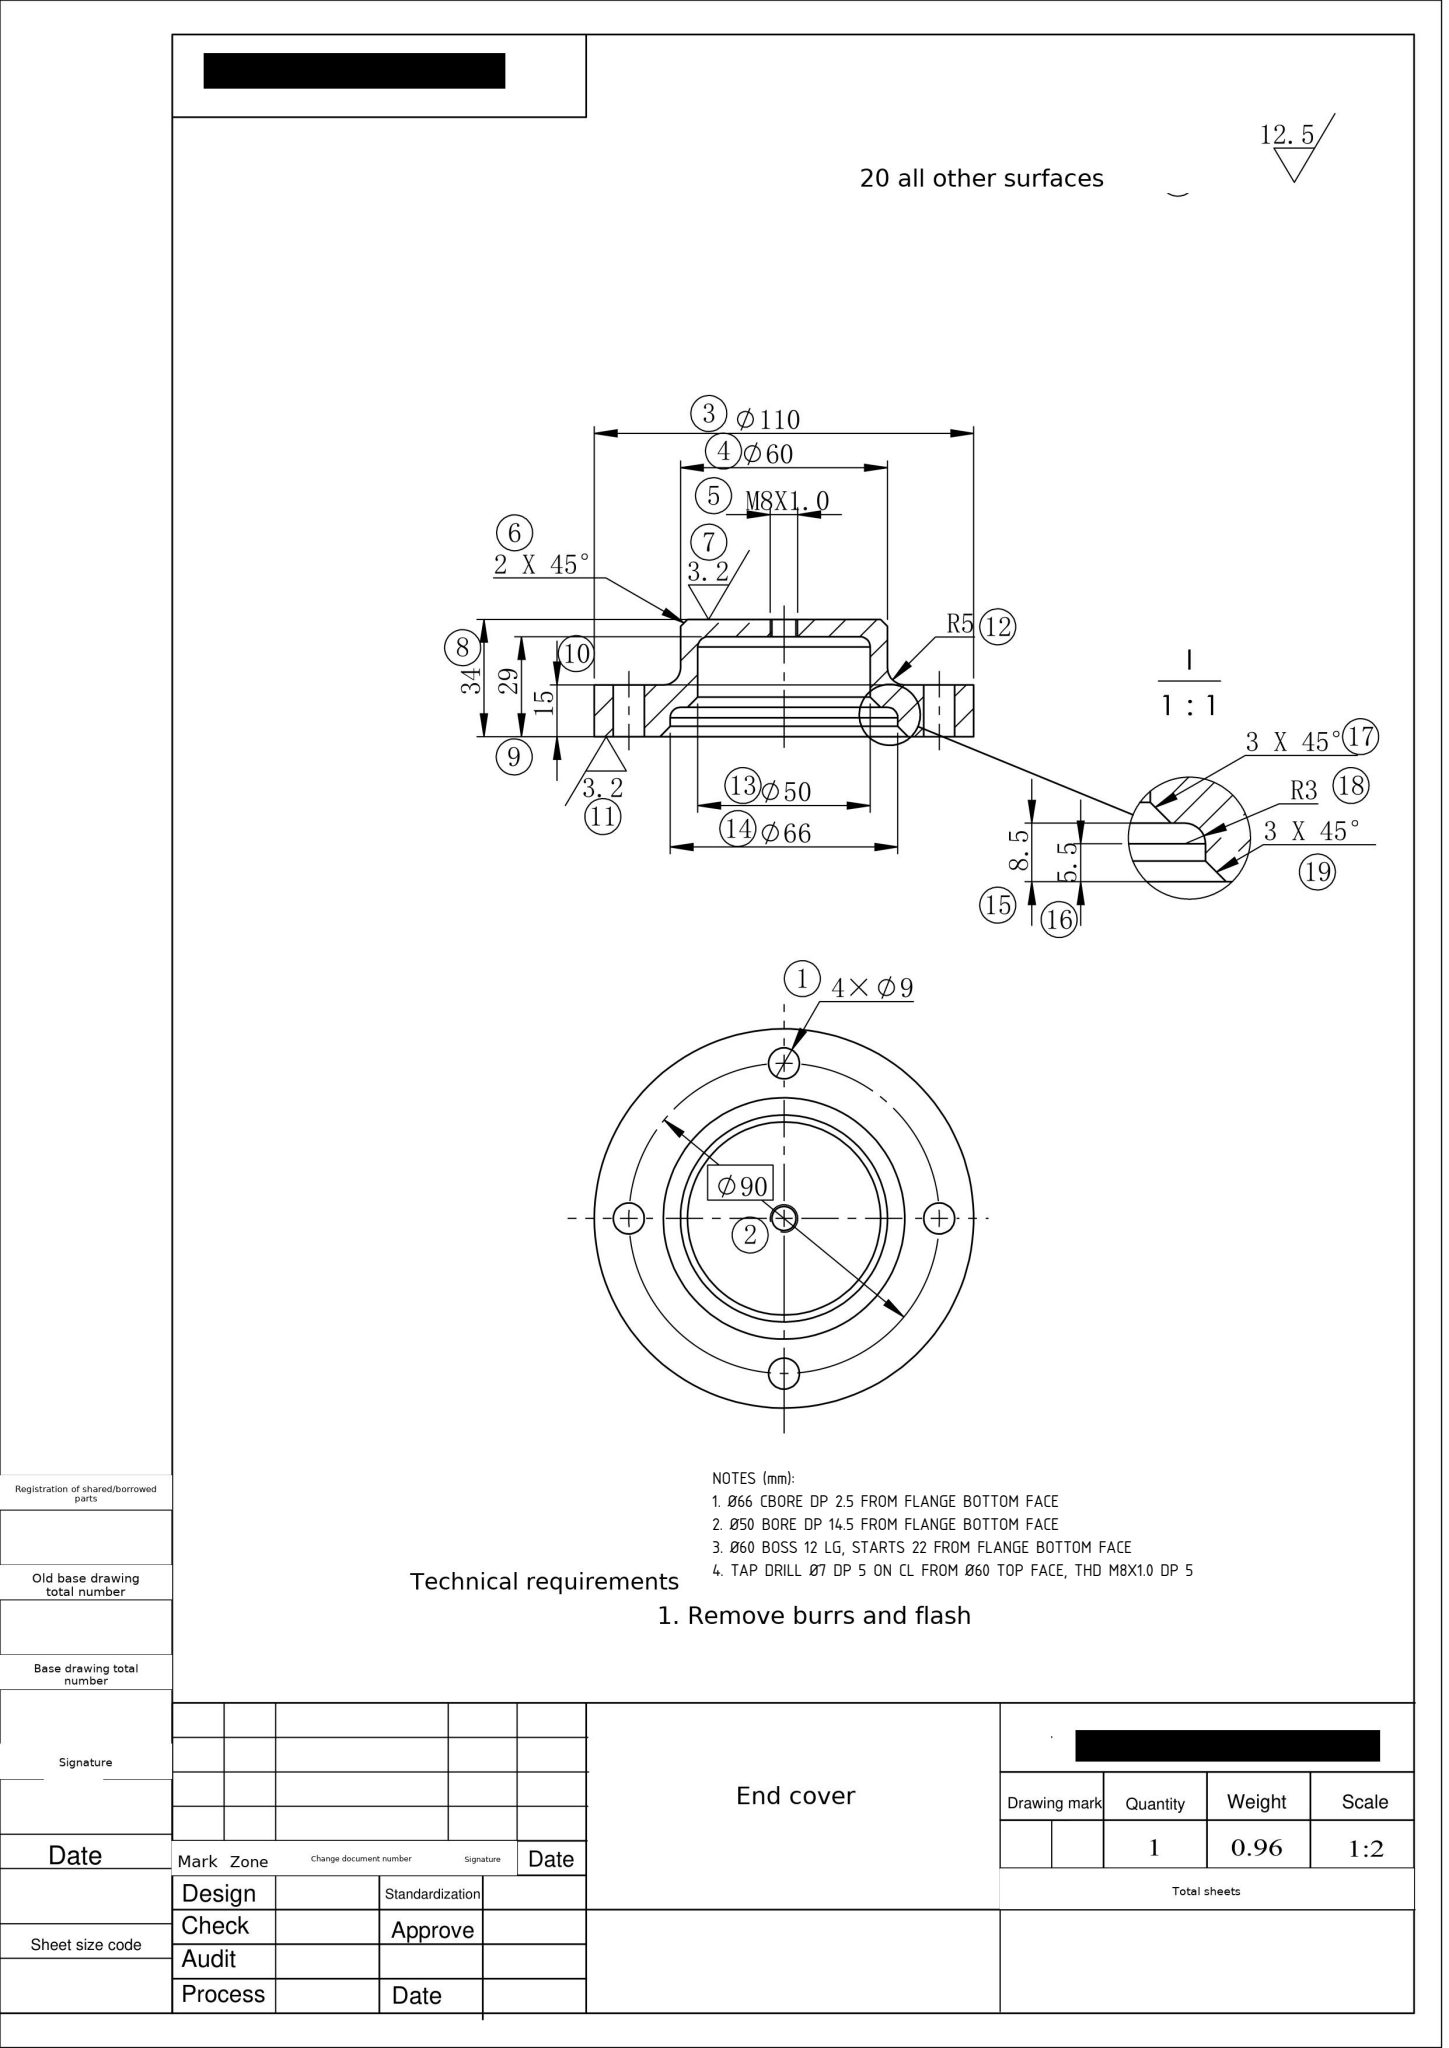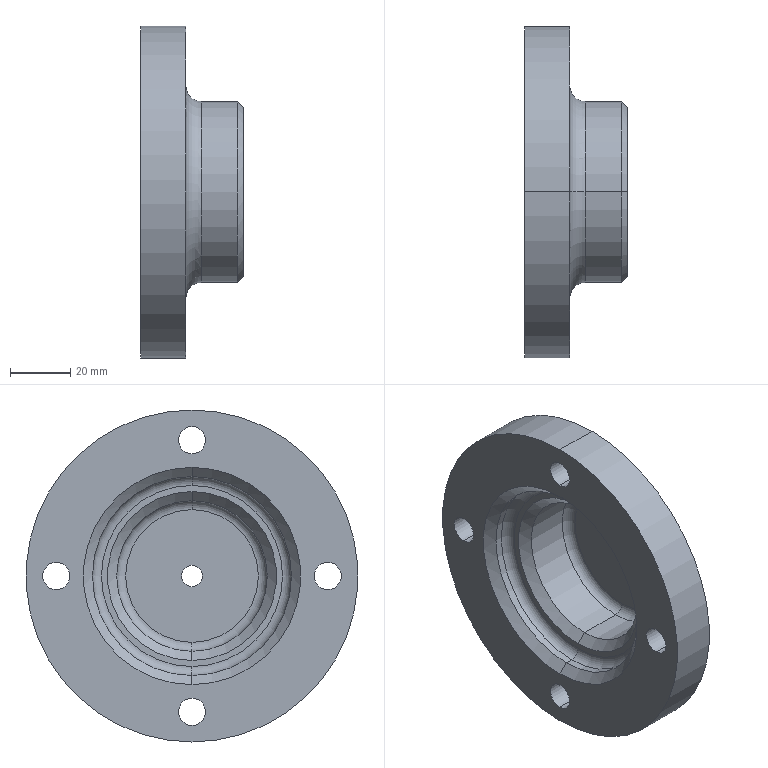Part | SolidWorks | mm | 1 solid | 35 faces | box 34 x 110 x 110 mm | volume 122601 mm3 | cylinder 18 | torus 6 | cone 6 | plane 5 | commonest cylinder face diameters 9 x8 7 x2 60 x2 50 x2 66 x2 110 x2
Drawing notes:
Ø66 CBORE DP 2.5 FROM FLANGE BOTTOM FACE | from the solid: cyl Ø66 axis x at (55,55), length 2.5 from x=0 (flange bottom face)
Ø50 BORE DP 14.5 FROM FLANGE BOTTOM FACE | from the solid: cyl Ø50 axis x at (55,55), length 14.5 from x=0 (flange bottom face)
Ø60 BOSS 12 LG, STARTS 22 FROM FLANGE BOTTOM FACE | from the solid: cyl Ø60 length 12 ending at top face x=34; start x=22; flange Ø110 face x=15
TAP DRILL Ø7 DP 5 ON CL FROM Ø60 TOP FACE, THD M8X1.0 DP 5 | from the solid: cyl Ø7 (M8x1.0 minor) axis x at (55,55), length 5.0, planes x=29 and x=34
STEP:
#1=CARTESIAN_POINT('',(-5.,0.,3.5));
#2=VERTEX_POINT('',#1);
#3=CARTESIAN_POINT('',(-5.,-0.,-3.5));
#4=VERTEX_POINT('',#3);
#5=CARTESIAN_POINT('',(-5.,0.,0.));
#6=DIRECTION('',(1.,0.,0.));
#7=DIRECTION('',(0.,-0.,-1.));
#8=AXIS2_PLACEMENT_3D('',#5,#6,#7);
#9=CIRCLE('',#8,3.5);
#10=EDGE_CURVE('',#2,#4,#9,.T.);
#11=ORIENTED_EDGE('',*,*,#10,.F.);
#12=CARTESIAN_POINT('',(0.,0.,3.5));
#13=VERTEX_POINT('',#12);
#14=CARTESIAN_POINT('',(0.,0.,3.5));
#15=DIRECTION('',(1.,0.,0.));
#16=VECTOR('',#15,1000.);
#17=LINE('',#14,#16);
#18=EDGE_CURVE('',#2,#13,#17,.T.);
#19=ORIENTED_EDGE('',*,*,#18,.T.);
#20=CARTESIAN_POINT('',(0.,-0.,-3.5));
#21=VERTEX_POINT('',#20);
#22=CARTESIAN_POINT('',(0.,0.,0.));
#23=DIRECTION('',(1.,0.,0.));
#24=DIRECTION('',(0.,-0.,-1.));
#25=AXIS2_PLACEMENT_3D('',#22,#23,#24);
#26=CIRCLE('',#25,3.5);
#27=EDGE_CURVE('',#13,#21,#26,.T.);
#28=ORIENTED_EDGE('',*,*,#27,.T.);
#29=CARTESIAN_POINT('',(0.,-0.,-3.5));
#30=DIRECTION('',(1.,0.,0.));
#31=VECTOR('',#30,1000.);
#32=LINE('',#29,#31);
#33=EDGE_CURVE('',#4,#21,#32,.T.);
#34=ORIENTED_EDGE('',*,*,#33,.F.);
#35=EDGE_LOOP('',(#11,#19,#28,#34));
#36=FACE_OUTER_BOUND('',#35,.T.);
#37=CARTESIAN_POINT('',(0.,0.,0.));
#38=DIRECTION('',(1.,0.,0.));
#39=DIRECTION('',(0.,-0.,-1.));
#40=AXIS2_PLACEMENT_3D('',#37,#38,#39);
#41=CYLINDRICAL_SURFACE('',#40,3.5);
#42=ADVANCED_FACE('',(#36),#41,.F.);
#43=CARTESIAN_POINT('',(-19.,0.,-49.5));
#44=VERTEX_POINT('',#43);
#45=CARTESIAN_POINT('',(-19.,0.,-40.5));
#46=VERTEX_POINT('',#45);
#47=CARTESIAN_POINT('',(-19.,0.,-45.));
#48=DIRECTION('',(-1.,0.,0.));
#49=DIRECTION('',(0.,0.,1.));
#50=AXIS2_PLACEMENT_3D('',#47,#48,#49);
#51=CIRCLE('',#50,4.5);
#52=EDGE_CURVE('',#44,#46,#51,.T.);
#53=ORIENTED_EDGE('',*,*,#52,.F.);
#54=CARTESIAN_POINT('',(-34.,0.,-49.5));
#55=VERTEX_POINT('',#54);
#56=CARTESIAN_POINT('',(-0.,0.,-49.5));
#57=DIRECTION('',(-1.,0.,0.));
#58=VECTOR('',#57,1000.);
#59=LINE('',#56,#58);
#60=EDGE_CURVE('',#44,#55,#59,.T.);
#61=ORIENTED_EDGE('',*,*,#60,.T.);
#62=CARTESIAN_POINT('',(-34.,0.,-40.5));
#63=VERTEX_POINT('',#62);
#64=CARTESIAN_POINT('',(-34.,0.,-45.));
#65=DIRECTION('',(-1.,0.,0.));
#66=DIRECTION('',(0.,0.,1.));
#67=AXIS2_PLACEMENT_3D('',#64,#65,#66);
#68=CIRCLE('',#67,4.5);
#69=EDGE_CURVE('',#55,#63,#68,.T.);
#70=ORIENTED_EDGE('',*,*,#69,.T.);
#71=CARTESIAN_POINT('',(-0.,0.,-40.5));
#72=DIRECTION('',(-1.,0.,0.));
#73=VECTOR('',#72,1000.);
#74=LINE('',#71,#73);
#75=EDGE_CURVE('',#46,#63,#74,.T.);
#76=ORIENTED_EDGE('',*,*,#75,.F.);
#77=EDGE_LOOP('',(#53,#61,#70,#76));
#78=FACE_OUTER_BOUND('',#77,.T.);
#79=CARTESIAN_POINT('',(-0.,0.,-45.));
#80=DIRECTION('',(-1.,0.,0.));
#81=DIRECTION('',(0.,0.,1.));
#82=AXIS2_PLACEMENT_3D('',#79,#80,#81);
#83=CYLINDRICAL_SURFACE('',#82,4.5);
#84=ADVANCED_FACE('',(#78),#83,.F.);
#85=CARTESIAN_POINT('',(-19.,-45.,-4.5));
#86=VERTEX_POINT('',#85);
#87=CARTESIAN_POINT('',(-19.,-45.,4.5));
#88=VERTEX_POINT('',#87);
#89=CARTESIAN_POINT('',(-19.,-45.,-0.));
#90=DIRECTION('',(-1.,0.,0.));
#91=DIRECTION('',(0.,0.,1.));
#92=AXIS2_PLACEMENT_3D('',#89,#90,#91);
#93=CIRCLE('',#92,4.5);
#94=EDGE_CURVE('',#86,#88,#93,.T.);
#95=ORIENTED_EDGE('',*,*,#94,.F.);
#96=CARTESIAN_POINT('',(-34.,-45.,-4.5));
#97=VERTEX_POINT('',#96);
#98=CARTESIAN_POINT('',(-0.,-45.,-4.5));
#99=DIRECTION('',(-1.,0.,0.));
#100=VECTOR('',#99,1000.);
#101=LINE('',#98,#100);
#102=EDGE_CURVE('',#86,#97,#101,.T.);
#103=ORIENTED_EDGE('',*,*,#102,.T.);
#104=CARTESIAN_POINT('',(-34.,-45.,4.5));
#105=VERTEX_POINT('',#104);
#106=CARTESIAN_POINT('',(-34.,-45.,-0.));
#107=DIRECTION('',(-1.,0.,0.));
#108=DIRECTION('',(0.,0.,1.));
#109=AXIS2_PLACEMENT_3D('',#106,#107,#108);
#110=CIRCLE('',#109,4.5);
#111=EDGE_CURVE('',#97,#105,#110,.T.);
#112=ORIENTED_EDGE('',*,*,#111,.T.);
#113=CARTESIAN_POINT('',(-0.,-45.,4.5));
#114=DIRECTION('',(-1.,0.,0.));
#115=VECTOR('',#114,1000.);
#116=LINE('',#113,#115);
#117=EDGE_CURVE('',#88,#105,#116,.T.);
#118=ORIENTED_EDGE('',*,*,#117,.F.);
#119=EDGE_LOOP('',(#95,#103,#112,#118));
#120=FACE_OUTER_BOUND('',#119,.T.);
#121=CARTESIAN_POINT('',(-0.,-45.,-0.));
#122=DIRECTION('',(-1.,0.,0.));
#123=DIRECTION('',(0.,0.,1.));
#124=AXIS2_PLACEMENT_3D('',#121,#122,#123);
#125=CYLINDRICAL_SURFACE('',#124,4.5);
#126=ADVANCED_FACE('',(#120),#125,.F.);
#127=CARTESIAN_POINT('',(-19.,-0.,40.5));
#128=VERTEX_POINT('',#127);
#129=CARTESIAN_POINT('',(-19.,-0.,49.5));
#130=VERTEX_POINT('',#129);
#131=CARTESIAN_POINT('',(-19.,-0.,45.));
#132=DIRECTION('',(-1.,0.,0.));
#133=DIRECTION('',(0.,0.,1.));
#134=AXIS2_PLACEMENT_3D('',#131,#132,#133);
#135=CIRCLE('',#134,4.5);
#136=EDGE_CURVE('',#128,#130,#135,.T.);
#137=ORIENTED_EDGE('',*,*,#136,.F.);
#138=CARTESIAN_POINT('',(-34.,-0.,40.5));
#139=VERTEX_POINT('',#138);
#140=CARTESIAN_POINT('',(-0.,-0.,40.5));
#141=DIRECTION('',(-1.,0.,0.));
#142=VECTOR('',#141,1000.);
#143=LINE('',#140,#142);
#144=EDGE_CURVE('',#128,#139,#143,.T.);
#145=ORIENTED_EDGE('',*,*,#144,.T.);
#146=CARTESIAN_POINT('',(-34.,-0.,49.5));
#147=VERTEX_POINT('',#146);
#148=CARTESIAN_POINT('',(-34.,-0.,45.));
#149=DIRECTION('',(-1.,0.,0.));
#150=DIRECTION('',(0.,0.,1.));
#151=AXIS2_PLACEMENT_3D('',#148,#149,#150);
#152=CIRCLE('',#151,4.5);
#153=EDGE_CURVE('',#139,#147,#152,.T.);
#154=ORIENTED_EDGE('',*,*,#153,.T.);
#155=CARTESIAN_POINT('',(-0.,-0.,49.5));
#156=DIRECTION('',(-1.,0.,0.));
#157=VECTOR('',#156,1000.);
#158=LINE('',#155,#157);
#159=EDGE_CURVE('',#130,#147,#158,.T.);
#160=ORIENTED_EDGE('',*,*,#159,.F.);
#161=EDGE_LOOP('',(#137,#145,#154,#160));
#162=FACE_OUTER_BOUND('',#161,.T.);
#163=CARTESIAN_POINT('',(-0.,-0.,45.));
#164=DIRECTION('',(-1.,0.,0.));
#165=DIRECTION('',(0.,0.,1.));
#166=AXIS2_PLACEMENT_3D('',#163,#164,#165);
#167=CYLINDRICAL_SURFACE('',#166,4.5);
#168=ADVANCED_FACE('',(#162),#167,.F.);
#169=CARTESIAN_POINT('',(-19.,45.,-4.5));
#170=VERTEX_POINT('',#169);
#171=CARTESIAN_POINT('',(-19.,45.,4.5));
#172=VERTEX_POINT('',#171);
#173=CARTESIAN_POINT('',(-19.,45.,0.));
#174=DIRECTION('',(-1.,0.,0.));
#175=DIRECTION('',(0.,0.,1.));
#176=AXIS2_PLACEMENT_3D('',#173,#174,#175);
#177=CIRCLE('',#176,4.5);
#178=EDGE_CURVE('',#170,#172,#177,.T.);
#179=ORIENTED_EDGE('',*,*,#178,.F.);
#180=CARTESIAN_POINT('',(-34.,45.,-4.5));
#181=VERTEX_POINT('',#180);
#182=CARTESIAN_POINT('',(-0.,45.,-4.5));
#183=DIRECTION('',(-1.,0.,0.));
#184=VECTOR('',#183,1000.);
#185=LINE('',#182,#184);
#186=EDGE_CURVE('',#170,#181,#185,.T.);
#187=ORIENTED_EDGE('',*,*,#186,.T.);
#188=CARTESIAN_POINT('',(-34.,45.,4.5));
#189=VERTEX_POINT('',#188);
#190=CARTESIAN_POINT('',(-34.,45.,0.));
#191=DIRECTION('',(-1.,0.,0.));
#192=DIRECTION('',(0.,0.,1.));
#193=AXIS2_PLACEMENT_3D('',#190,#191,#192);
#194=CIRCLE('',#193,4.5);
#195=EDGE_CURVE('',#181,#189,#194,.T.);
#196=ORIENTED_EDGE('',*,*,#195,.T.);
#197=CARTESIAN_POINT('',(-0.,45.,4.5));
#198=DIRECTION('',(-1.,0.,0.));
#199=VECTOR('',#198,1000.);
#200=LINE('',#197,#199);
#201=EDGE_CURVE('',#172,#189,#200,.T.);
#202=ORIENTED_EDGE('',*,*,#201,.F.);
#203=EDGE_LOOP('',(#179,#187,#196,#202));
#204=FACE_OUTER_BOUND('',#203,.T.);
#205=CARTESIAN_POINT('',(-0.,45.,0.));
#206=DIRECTION('',(-1.,0.,0.));
#207=DIRECTION('',(0.,0.,1.));
#208=AXIS2_PLACEMENT_3D('',#205,#206,#207);
#209=CYLINDRICAL_SURFACE('',#208,4.5);
#210=ADVANCED_FACE('',(#204),#209,.F.);
#211=CARTESIAN_POINT('',(-19.,0.,-35.));
#212=VERTEX_POINT('',#211);
#213=CARTESIAN_POINT('',(-19.,0.,35.));
#214=VERTEX_POINT('',#213);
#215=CARTESIAN_POINT('',(-19.,0.,0.));
#216=DIRECTION('',(-1.,0.,0.));
#217=DIRECTION('',(0.,0.,1.));
#218=AXIS2_PLACEMENT_3D('',#215,#216,#217);
#219=CIRCLE('',#218,35.);
#220=EDGE_CURVE('',#212,#214,#219,.T.);
#221=ORIENTED_EDGE('',*,*,#220,.F.);
#222=CARTESIAN_POINT('',(-14.,0.,-30.));
#223=VERTEX_POINT('',#222);
#224=CARTESIAN_POINT('',(-14.,0.,-35.));
#225=DIRECTION('',(0.,1.,0.));
#226=DIRECTION('',(0.,-0.,1.));
#227=AXIS2_PLACEMENT_3D('',#224,#225,#226);
#228=CIRCLE('',#227,5.);
#229=EDGE_CURVE('',#212,#223,#228,.T.);
#230=ORIENTED_EDGE('',*,*,#229,.T.);
#231=CARTESIAN_POINT('',(-14.,0.,30.));
#232=VERTEX_POINT('',#231);
#233=CARTESIAN_POINT('',(-14.,0.,0.));
#234=DIRECTION('',(-1.,0.,0.));
#235=DIRECTION('',(0.,0.,1.));
#236=AXIS2_PLACEMENT_3D('',#233,#234,#235);
#237=CIRCLE('',#236,30.);
#238=EDGE_CURVE('',#223,#232,#237,.T.);
#239=ORIENTED_EDGE('',*,*,#238,.T.);
#240=CARTESIAN_POINT('',(-14.,0.,35.));
#241=DIRECTION('',(0.,-1.,0.));
#242=DIRECTION('',(0.,-0.,-1.));
#243=AXIS2_PLACEMENT_3D('',#240,#241,#242);
#244=CIRCLE('',#243,5.);
#245=EDGE_CURVE('',#214,#232,#244,.T.);
#246=ORIENTED_EDGE('',*,*,#245,.F.);
#247=EDGE_LOOP('',(#221,#230,#239,#246));
#248=FACE_OUTER_BOUND('',#247,.T.);
#249=CARTESIAN_POINT('',(-14.,0.,0.));
#250=DIRECTION('',(-1.,0.,0.));
#251=DIRECTION('',(0.,0.,1.));
#252=AXIS2_PLACEMENT_3D('',#249,#250,#251);
#253=TOROIDAL_SURFACE('',#252,35.,5.);
#254=ADVANCED_FACE('',(#248),#253,.F.);
#255=CARTESIAN_POINT('',(-2.,0.,30.));
#256=VERTEX_POINT('',#255);
#257=CARTESIAN_POINT('',(-2.,0.,-30.));
#258=VERTEX_POINT('',#257);
#259=CARTESIAN_POINT('',(-2.,0.,0.));
#260=DIRECTION('',(-1.,0.,0.));
#261=DIRECTION('',(0.,0.,1.));
#262=AXIS2_PLACEMENT_3D('',#259,#260,#261);
#263=CIRCLE('',#262,30.);
#264=EDGE_CURVE('',#256,#258,#263,.T.);
#265=ORIENTED_EDGE('',*,*,#264,.T.);
#266=CARTESIAN_POINT('',(-65.563,0.,-30.));
#267=DIRECTION('',(-1.,0.,0.));
#268=VECTOR('',#267,1000.);
#269=LINE('',#266,#268);
#270=EDGE_CURVE('',#258,#223,#269,.T.);
#271=ORIENTED_EDGE('',*,*,#270,.T.);
#272=CARTESIAN_POINT('',(-14.,0.,0.));
#273=DIRECTION('',(-1.,0.,0.));
#274=DIRECTION('',(0.,0.,1.));
#275=AXIS2_PLACEMENT_3D('',#272,#273,#274);
#276=CIRCLE('',#275,30.);
#277=EDGE_CURVE('',#232,#223,#276,.T.);
#278=ORIENTED_EDGE('',*,*,#277,.F.);
#279=CARTESIAN_POINT('',(-65.563,0.,30.));
#280=DIRECTION('',(-1.,0.,0.));
#281=VECTOR('',#280,1000.);
#282=LINE('',#279,#281);
#283=EDGE_CURVE('',#256,#232,#282,.T.);
#284=ORIENTED_EDGE('',*,*,#283,.F.);
#285=EDGE_LOOP('',(#265,#271,#278,#284));
#286=FACE_OUTER_BOUND('',#285,.T.);
#287=CARTESIAN_POINT('',(-65.563,0.,0.));
#288=DIRECTION('',(-1.,0.,0.));
#289=DIRECTION('',(0.,0.,1.));
#290=AXIS2_PLACEMENT_3D('',#287,#288,#289);
#291=CYLINDRICAL_SURFACE('',#290,30.);
#292=ADVANCED_FACE('',(#286),#291,.T.);
#293=CARTESIAN_POINT('',(-0.,0.,28.));
#294=VERTEX_POINT('',#293);
#295=CARTESIAN_POINT('',(-0.,0.,-28.));
#296=VERTEX_POINT('',#295);
#297=CARTESIAN_POINT('',(-0.,0.,0.));
#298=DIRECTION('',(-1.,0.,0.));
#299=DIRECTION('',(0.,0.,1.));
#300=AXIS2_PLACEMENT_3D('',#297,#298,#299);
#301=CIRCLE('',#300,28.);
#302=EDGE_CURVE('',#294,#296,#301,.T.);
#303=ORIENTED_EDGE('',*,*,#302,.T.);
#304=CARTESIAN_POINT('',(-0.,0.,-28.));
#305=DIRECTION('',(-0.7071,0.,-0.7071));
#306=VECTOR('',#305,1000.);
#307=LINE('',#304,#306);
#308=EDGE_CURVE('',#296,#258,#307,.T.);
#309=ORIENTED_EDGE('',*,*,#308,.T.);
#310=ORIENTED_EDGE('',*,*,#264,.F.);
#311=CARTESIAN_POINT('',(-0.,0.,28.));
#312=DIRECTION('',(-0.7071,0.,0.7071));
#313=VECTOR('',#312,1000.);
#314=LINE('',#311,#313);
#315=EDGE_CURVE('',#294,#256,#314,.T.);
#316=ORIENTED_EDGE('',*,*,#315,.F.);
#317=EDGE_LOOP('',(#303,#309,#310,#316));
#318=FACE_OUTER_BOUND('',#317,.T.);
#319=CARTESIAN_POINT('',(-0.,0.,0.));
#320=DIRECTION('',(-1.,0.,0.));
#321=DIRECTION('',(0.,0.,1.));
#322=AXIS2_PLACEMENT_3D('',#319,#320,#321);
#323=CONICAL_SURFACE('',#322,28.,0.7854);
#324=ADVANCED_FACE('',(#318),#323,.T.);
#325=CARTESIAN_POINT('',(-5.,0.,-22.));
#326=VERTEX_POINT('',#325);
#327=CARTESIAN_POINT('',(-5.,0.,22.));
#328=VERTEX_POINT('',#327);
#329=CARTESIAN_POINT('',(-5.,0.,0.));
#330=DIRECTION('',(-1.,0.,0.));
#331=DIRECTION('',(0.,0.,1.));
#332=AXIS2_PLACEMENT_3D('',#329,#330,#331);
#333=CIRCLE('',#332,22.);
#334=EDGE_CURVE('',#326,#328,#333,.T.);
#335=ORIENTED_EDGE('',*,*,#334,.F.);
#336=CARTESIAN_POINT('',(-8.,0.,-25.));
#337=VERTEX_POINT('',#336);
#338=CARTESIAN_POINT('',(-8.,0.,-22.));
#339=DIRECTION('',(0.,1.,0.));
#340=DIRECTION('',(0.,-0.,1.));
#341=AXIS2_PLACEMENT_3D('',#338,#339,#340);
#342=CIRCLE('',#341,3.);
#343=EDGE_CURVE('',#326,#337,#342,.T.);
#344=ORIENTED_EDGE('',*,*,#343,.T.);
#345=CARTESIAN_POINT('',(-8.,0.,25.));
#346=VERTEX_POINT('',#345);
#347=CARTESIAN_POINT('',(-8.,0.,0.));
#348=DIRECTION('',(-1.,0.,0.));
#349=DIRECTION('',(0.,0.,1.));
#350=AXIS2_PLACEMENT_3D('',#347,#348,#349);
#351=CIRCLE('',#350,25.);
#352=EDGE_CURVE('',#337,#346,#351,.T.);
#353=ORIENTED_EDGE('',*,*,#352,.T.);
#354=CARTESIAN_POINT('',(-8.,0.,22.));
#355=DIRECTION('',(0.,-1.,0.));
#356=DIRECTION('',(0.,-0.,-1.));
#357=AXIS2_PLACEMENT_3D('',#354,#355,#356);
#358=CIRCLE('',#357,3.);
#359=EDGE_CURVE('',#328,#346,#358,.T.);
#360=ORIENTED_EDGE('',*,*,#359,.F.);
#361=EDGE_LOOP('',(#335,#344,#353,#360));
#362=FACE_OUTER_BOUND('',#361,.T.);
#363=CARTESIAN_POINT('',(-8.,0.,0.));
#364=DIRECTION('',(-1.,0.,0.));
#365=DIRECTION('',(0.,0.,1.));
#366=AXIS2_PLACEMENT_3D('',#363,#364,#365);
#367=TOROIDAL_SURFACE('',#366,22.,3.);
#368=ADVANCED_FACE('',(#362),#367,.F.);
#369=ORIENTED_EDGE('',*,*,#352,.F.);
#370=CARTESIAN_POINT('',(-22.5,0.,-25.));
#371=VERTEX_POINT('',#370);
#372=CARTESIAN_POINT('',(-65.563,0.,-25.));
#373=DIRECTION('',(-1.,0.,0.));
#374=VECTOR('',#373,1000.);
#375=LINE('',#372,#374);
#376=EDGE_CURVE('',#337,#371,#375,.T.);
#377=ORIENTED_EDGE('',*,*,#376,.T.);
#378=CARTESIAN_POINT('',(-22.5,0.,25.));
#379=VERTEX_POINT('',#378);
#380=CARTESIAN_POINT('',(-22.5,0.,0.));
#381=DIRECTION('',(-1.,0.,0.));
#382=DIRECTION('',(0.,0.,1.));
#383=AXIS2_PLACEMENT_3D('',#380,#381,#382);
#384=CIRCLE('',#383,25.);
#385=EDGE_CURVE('',#371,#379,#384,.T.);
#386=ORIENTED_EDGE('',*,*,#385,.T.);
#387=CARTESIAN_POINT('',(-65.563,0.,25.));
#388=DIRECTION('',(-1.,0.,0.));
#389=VECTOR('',#388,1000.);
#390=LINE('',#387,#389);
#391=EDGE_CURVE('',#346,#379,#390,.T.);
#392=ORIENTED_EDGE('',*,*,#391,.F.);
#393=EDGE_LOOP('',(#369,#377,#386,#392));
#394=FACE_OUTER_BOUND('',#393,.T.);
#395=CARTESIAN_POINT('',(-65.563,0.,0.));
#396=DIRECTION('',(-1.,0.,0.));
#397=DIRECTION('',(0.,0.,1.));
#398=AXIS2_PLACEMENT_3D('',#395,#396,#397);
#399=CYLINDRICAL_SURFACE('',#398,25.);
#400=ADVANCED_FACE('',(#394),#399,.F.);
#401=ORIENTED_EDGE('',*,*,#385,.F.);
#402=CARTESIAN_POINT('',(-25.5,0.,-28.));
#403=VERTEX_POINT('',#402);
#404=CARTESIAN_POINT('',(-25.5,0.,-28.));
#405=DIRECTION('',(-0.7071,0.,-0.7071));
#406=VECTOR('',#405,1000.);
#407=LINE('',#404,#406);
#408=EDGE_CURVE('',#371,#403,#407,.T.);
#409=ORIENTED_EDGE('',*,*,#408,.T.);
#410=CARTESIAN_POINT('',(-25.5,0.,28.));
#411=VERTEX_POINT('',#410);
#412=CARTESIAN_POINT('',(-25.5,0.,0.));
#413=DIRECTION('',(-1.,0.,0.));
#414=DIRECTION('',(0.,0.,1.));
#415=AXIS2_PLACEMENT_3D('',#412,#413,#414);
#416=CIRCLE('',#415,28.);
#417=EDGE_CURVE('',#403,#411,#416,.T.);
#418=ORIENTED_EDGE('',*,*,#417,.T.);
#419=CARTESIAN_POINT('',(-25.5,0.,28.));
#420=DIRECTION('',(-0.7071,0.,0.7071));
#421=VECTOR('',#420,1000.);
#422=LINE('',#419,#421);
#423=EDGE_CURVE('',#379,#411,#422,.T.);
#424=ORIENTED_EDGE('',*,*,#423,.F.);
#425=EDGE_LOOP('',(#401,#409,#418,#424));
#426=FACE_OUTER_BOUND('',#425,.T.);
#427=CARTESIAN_POINT('',(-25.5,0.,0.));
#428=DIRECTION('',(-1.,0.,0.));
#429=DIRECTION('',(0.,0.,1.));
#430=AXIS2_PLACEMENT_3D('',#427,#428,#429);
#431=CONICAL_SURFACE('',#430,28.,0.7854);
#432=ADVANCED_FACE('',(#426),#431,.F.);
#433=CARTESIAN_POINT('',(-25.5,0.,-30.));
#434=VERTEX_POINT('',#433);
#435=CARTESIAN_POINT('',(-25.5,0.,30.));
#436=VERTEX_POINT('',#435);
#437=CARTESIAN_POINT('',(-25.5,0.,0.));
#438=DIRECTION('',(-1.,0.,0.));
#439=DIRECTION('',(0.,0.,1.));
#440=AXIS2_PLACEMENT_3D('',#437,#438,#439);
#441=CIRCLE('',#440,30.);
#442=EDGE_CURVE('',#434,#436,#441,.T.);
#443=ORIENTED_EDGE('',*,*,#442,.F.);
#444=CARTESIAN_POINT('',(-28.5,0.,-33.));
#445=VERTEX_POINT('',#444);
#446=CARTESIAN_POINT('',(-28.5,0.,-30.));
#447=DIRECTION('',(0.,1.,0.));
#448=DIRECTION('',(0.,-0.,1.));
#449=AXIS2_PLACEMENT_3D('',#446,#447,#448);
#450=CIRCLE('',#449,3.);
#451=EDGE_CURVE('',#434,#445,#450,.T.);
#452=ORIENTED_EDGE('',*,*,#451,.T.);
#453=CARTESIAN_POINT('',(-28.5,0.,33.));
#454=VERTEX_POINT('',#453);
#455=CARTESIAN_POINT('',(-28.5,0.,0.));
#456=DIRECTION('',(-1.,0.,0.));
#457=DIRECTION('',(0.,0.,1.));
#458=AXIS2_PLACEMENT_3D('',#455,#456,#457);
#459=CIRCLE('',#458,33.);
#460=EDGE_CURVE('',#445,#454,#459,.T.);
#461=ORIENTED_EDGE('',*,*,#460,.T.);
#462=CARTESIAN_POINT('',(-28.5,0.,30.));
#463=DIRECTION('',(0.,-1.,0.));
#464=DIRECTION('',(0.,-0.,-1.));
#465=AXIS2_PLACEMENT_3D('',#462,#463,#464);
#466=CIRCLE('',#465,3.);
#467=EDGE_CURVE('',#436,#454,#466,.T.);
#468=ORIENTED_EDGE('',*,*,#467,.F.);
#469=EDGE_LOOP('',(#443,#452,#461,#468));
#470=FACE_OUTER_BOUND('',#469,.T.);
#471=CARTESIAN_POINT('',(-28.5,0.,0.));
#472=DIRECTION('',(-1.,0.,0.));
#473=DIRECTION('',(0.,0.,1.));
#474=AXIS2_PLACEMENT_3D('',#471,#472,#473);
#475=TOROIDAL_SURFACE('',#474,30.,3.);
#476=ADVANCED_FACE('',(#470),#475,.F.);
#477=ORIENTED_EDGE('',*,*,#460,.F.);
#478=CARTESIAN_POINT('',(-31.,0.,-33.));
#479=VERTEX_POINT('',#478);
#480=CARTESIAN_POINT('',(-65.563,0.,-33.));
#481=DIRECTION('',(-1.,0.,0.));
#482=VECTOR('',#481,1000.);
#483=LINE('',#480,#482);
#484=EDGE_CURVE('',#445,#479,#483,.T.);
#485=ORIENTED_EDGE('',*,*,#484,.T.);
#486=CARTESIAN_POINT('',(-31.,0.,33.));
#487=VERTEX_POINT('',#486);
#488=CARTESIAN_POINT('',(-31.,0.,0.));
#489=DIRECTION('',(-1.,0.,0.));
#490=DIRECTION('',(0.,0.,1.));
#491=AXIS2_PLACEMENT_3D('',#488,#489,#490);
#492=CIRCLE('',#491,33.);
#493=EDGE_CURVE('',#479,#487,#492,.T.);
#494=ORIENTED_EDGE('',*,*,#493,.T.);
#495=CARTESIAN_POINT('',(-65.563,0.,33.));
#496=DIRECTION('',(-1.,0.,0.));
#497=VECTOR('',#496,1000.);
#498=LINE('',#495,#497);
#499=EDGE_CURVE('',#454,#487,#498,.T.);
#500=ORIENTED_EDGE('',*,*,#499,.F.);
#501=EDGE_LOOP('',(#477,#485,#494,#500));
#502=FACE_OUTER_BOUND('',#501,.T.);
#503=CARTESIAN_POINT('',(-65.563,0.,0.));
#504=DIRECTION('',(-1.,0.,0.));
#505=DIRECTION('',(0.,0.,1.));
#506=AXIS2_PLACEMENT_3D('',#503,#504,#505);
#507=CYLINDRICAL_SURFACE('',#506,33.);
#508=ADVANCED_FACE('',(#502),#507,.F.);
#509=ORIENTED_EDGE('',*,*,#493,.F.);
#510=CARTESIAN_POINT('',(-34.,0.,-36.));
#511=VERTEX_POINT('',#510);
#512=CARTESIAN_POINT('',(-34.,0.,-36.));
#513=DIRECTION('',(-0.7071,0.,-0.7071));
#514=VECTOR('',#513,1000.);
#515=LINE('',#512,#514);
#516=EDGE_CURVE('',#479,#511,#515,.T.);
#517=ORIENTED_EDGE('',*,*,#516,.T.);
#518=CARTESIAN_POINT('',(-34.,0.,36.));
#519=VERTEX_POINT('',#518);
#520=CARTESIAN_POINT('',(-34.,0.,0.));
#521=DIRECTION('',(-1.,0.,0.));
#522=DIRECTION('',(0.,0.,1.));
#523=AXIS2_PLACEMENT_3D('',#520,#521,#522);
#524=CIRCLE('',#523,36.);
#525=EDGE_CURVE('',#511,#519,#524,.T.);
#526=ORIENTED_EDGE('',*,*,#525,.T.);
#527=CARTESIAN_POINT('',(-34.,0.,36.));
#528=DIRECTION('',(-0.7071,0.,0.7071));
#529=VECTOR('',#528,1000.);
#530=LINE('',#527,#529);
#531=EDGE_CURVE('',#487,#519,#530,.T.);
#532=ORIENTED_EDGE('',*,*,#531,.F.);
#533=EDGE_LOOP('',(#509,#517,#526,#532));
#534=FACE_OUTER_BOUND('',#533,.T.);
#535=CARTESIAN_POINT('',(-34.,0.,0.));
#536=DIRECTION('',(-1.,0.,0.));
#537=DIRECTION('',(0.,0.,1.));
#538=AXIS2_PLACEMENT_3D('',#535,#536,#537);
#539=CONICAL_SURFACE('',#538,36.,0.7854);
#540=ADVANCED_FACE('',(#534),#539,.F.);
#541=CARTESIAN_POINT('',(-19.,0.,55.));
#542=VERTEX_POINT('',#541);
#543=CARTESIAN_POINT('',(-19.,0.,-55.));
#544=VERTEX_POINT('',#543);
#545=CARTESIAN_POINT('',(-19.,0.,0.));
#546=DIRECTION('',(-1.,0.,0.));
#547=DIRECTION('',(0.,0.,1.));
#548=AXIS2_PLACEMENT_3D('',#545,#546,#547);
#549=CIRCLE('',#548,55.);
#550=EDGE_CURVE('',#542,#544,#549,.T.);
#551=ORIENTED_EDGE('',*,*,#550,.T.);
#552=CARTESIAN_POINT('',(-34.,0.,-55.));
#553=VERTEX_POINT('',#552);
#554=CARTESIAN_POINT('',(-65.563,0.,-55.));
#555=DIRECTION('',(-1.,0.,0.));
#556=VECTOR('',#555,1000.);
#557=LINE('',#554,#556);
#558=EDGE_CURVE('',#544,#553,#557,.T.);
#559=ORIENTED_EDGE('',*,*,#558,.T.);
#560=CARTESIAN_POINT('',(-34.,0.,55.));
#561=VERTEX_POINT('',#560);
#562=CARTESIAN_POINT('',(-34.,0.,0.));
#563=DIRECTION('',(-1.,0.,0.));
#564=DIRECTION('',(0.,0.,1.));
#565=AXIS2_PLACEMENT_3D('',#562,#563,#564);
#566=CIRCLE('',#565,55.);
#567=EDGE_CURVE('',#561,#553,#566,.T.);
#568=ORIENTED_EDGE('',*,*,#567,.F.);
#569=CARTESIAN_POINT('',(-65.563,0.,55.));
#570=DIRECTION('',(-1.,0.,0.));
#571=VECTOR('',#570,1000.);
#572=LINE('',#569,#571);
#573=EDGE_CURVE('',#542,#561,#572,.T.);
#574=ORIENTED_EDGE('',*,*,#573,.F.);
#575=EDGE_LOOP('',(#551,#559,#568,#574));
#576=FACE_OUTER_BOUND('',#575,.T.);
#577=CARTESIAN_POINT('',(-65.563,0.,0.));
#578=DIRECTION('',(-1.,0.,0.));
#579=DIRECTION('',(0.,0.,1.));
#580=AXIS2_PLACEMENT_3D('',#577,#578,#579);
#581=CYLINDRICAL_SURFACE('',#580,55.);
#582=ADVANCED_FACE('',(#576),#581,.T.);
#583=ORIENTED_EDGE('',*,*,#558,.F.);
#584=CARTESIAN_POINT('',(-19.,0.,0.));
#585=DIRECTION('',(-1.,0.,0.));
#586=DIRECTION('',(0.,0.,1.));
#587=AXIS2_PLACEMENT_3D('',#584,#585,#586);
#588=CIRCLE('',#587,55.);
#589=EDGE_CURVE('',#544,#542,#588,.T.);
#590=ORIENTED_EDGE('',*,*,#589,.T.);
#591=ORIENTED_EDGE('',*,*,#573,.T.);
#592=CARTESIAN_POINT('',(-34.,0.,0.));
#593=DIRECTION('',(-1.,0.,0.));
#594=DIRECTION('',(0.,0.,1.));
#595=AXIS2_PLACEMENT_3D('',#592,#593,#594);
#596=CIRCLE('',#595,55.);
#597=EDGE_CURVE('',#553,#561,#596,.T.);
#598=ORIENTED_EDGE('',*,*,#597,.F.);
#599=EDGE_LOOP('',(#583,#590,#591,#598));
#600=FACE_OUTER_BOUND('',#599,.T.);
#601=CARTESIAN_POINT('',(-65.563,0.,0.));
#602=DIRECTION('',(-1.,0.,0.));
#603=DIRECTION('',(0.,0.,1.));
#604=AXIS2_PLACEMENT_3D('',#601,#602,#603);
#605=CYLINDRICAL_SURFACE('',#604,55.);
#606=ADVANCED_FACE('',(#600),#605,.T.);
#607=CARTESIAN_POINT('',(-34.,0.,-45.));
#608=DIRECTION('',(-1.,0.,0.));
#609=DIRECTION('',(0.,0.,1.));
#610=AXIS2_PLACEMENT_3D('',#607,#608,#609);
#611=CIRCLE('',#610,4.5);
#612=EDGE_CURVE('',#63,#55,#611,.T.);
#613=ORIENTED_EDGE('',*,*,#612,.F.);
#614=ORIENTED_EDGE('',*,*,#69,.F.);
#615=EDGE_LOOP('',(#613,#614));
#616=FACE_BOUND('',#615,.T.);
#617=CARTESIAN_POINT('',(-34.,-45.,-0.));
#618=DIRECTION('',(-1.,0.,0.));
#619=DIRECTION('',(0.,0.,1.));
#620=AXIS2_PLACEMENT_3D('',#617,#618,#619);
#621=CIRCLE('',#620,4.5);
#622=EDGE_CURVE('',#105,#97,#621,.T.);
#623=ORIENTED_EDGE('',*,*,#622,.F.);
#624=ORIENTED_EDGE('',*,*,#111,.F.);
#625=EDGE_LOOP('',(#623,#624));
#626=FACE_BOUND('',#625,.T.);
#627=CARTESIAN_POINT('',(-34.,-0.,45.));
#628=DIRECTION('',(-1.,0.,0.));
#629=DIRECTION('',(0.,0.,1.));
#630=AXIS2_PLACEMENT_3D('',#627,#628,#629);
#631=CIRCLE('',#630,4.5);
#632=EDGE_CURVE('',#147,#139,#631,.T.);
#633=ORIENTED_EDGE('',*,*,#632,.F.);
#634=ORIENTED_EDGE('',*,*,#153,.F.);
#635=EDGE_LOOP('',(#633,#634));
#636=FACE_BOUND('',#635,.T.);
#637=CARTESIAN_POINT('',(-34.,45.,0.));
#638=DIRECTION('',(-1.,0.,0.));
#639=DIRECTION('',(0.,0.,1.));
#640=AXIS2_PLACEMENT_3D('',#637,#638,#639);
#641=CIRCLE('',#640,4.5);
#642=EDGE_CURVE('',#189,#181,#641,.T.);
#643=ORIENTED_EDGE('',*,*,#642,.F.);
#644=ORIENTED_EDGE('',*,*,#195,.F.);
#645=EDGE_LOOP('',(#643,#644));
#646=FACE_BOUND('',#645,.T.);
#647=CARTESIAN_POINT('',(-34.,0.,0.));
#648=DIRECTION('',(-1.,0.,0.));
#649=DIRECTION('',(0.,0.,1.));
#650=AXIS2_PLACEMENT_3D('',#647,#648,#649);
#651=CIRCLE('',#650,36.);
#652=EDGE_CURVE('',#519,#511,#651,.T.);
#653=ORIENTED_EDGE('',*,*,#652,.F.);
#654=ORIENTED_EDGE('',*,*,#525,.F.);
#655=EDGE_LOOP('',(#653,#654));
#656=FACE_BOUND('',#655,.T.);
#657=ORIENTED_EDGE('',*,*,#567,.T.);
#658=ORIENTED_EDGE('',*,*,#597,.T.);
#659=EDGE_LOOP('',(#657,#658));
#660=FACE_OUTER_BOUND('',#659,.T.);
#661=CARTESIAN_POINT('',(-34.,55.,0.));
#662=DIRECTION('',(1.,0.,0.));
#663=DIRECTION('',(0.,-0.,-1.));
#664=AXIS2_PLACEMENT_3D('',#661,#662,#663);
#665=PLANE('',#664);
#666=ADVANCED_FACE('',(#616,#626,#636,#646,#656,#660),#665,.F.);
#667=ORIENTED_EDGE('',*,*,#516,.F.);
#668=CARTESIAN_POINT('',(-31.,0.,0.));
#669=DIRECTION('',(-1.,0.,0.));
#670=DIRECTION('',(0.,0.,1.));
#671=AXIS2_PLACEMENT_3D('',#668,#669,#670);
#672=CIRCLE('',#671,33.);
#673=EDGE_CURVE('',#487,#479,#672,.T.);
#674=ORIENTED_EDGE('',*,*,#673,.F.);
#675=ORIENTED_EDGE('',*,*,#531,.T.);
#676=ORIENTED_EDGE('',*,*,#652,.T.);
#677=EDGE_LOOP('',(#667,#674,#675,#676));
#678=FACE_OUTER_BOUND('',#677,.T.);
#679=CARTESIAN_POINT('',(-34.,0.,0.));
#680=DIRECTION('',(-1.,0.,0.));
#681=DIRECTION('',(0.,0.,1.));
#682=AXIS2_PLACEMENT_3D('',#679,#680,#681);
#683=CONICAL_SURFACE('',#682,36.,0.7854);
#684=ADVANCED_FACE('',(#678),#683,.F.);
#685=ORIENTED_EDGE('',*,*,#484,.F.);
#686=CARTESIAN_POINT('',(-28.5,0.,0.));
#687=DIRECTION('',(-1.,0.,0.));
#688=DIRECTION('',(0.,0.,1.));
#689=AXIS2_PLACEMENT_3D('',#686,#687,#688);
#690=CIRCLE('',#689,33.);
#691=EDGE_CURVE('',#454,#445,#690,.T.);
#692=ORIENTED_EDGE('',*,*,#691,.F.);
#693=ORIENTED_EDGE('',*,*,#499,.T.);
#694=ORIENTED_EDGE('',*,*,#673,.T.);
#695=EDGE_LOOP('',(#685,#692,#693,#694));
#696=FACE_OUTER_BOUND('',#695,.T.);
#697=CARTESIAN_POINT('',(-65.563,0.,0.));
#698=DIRECTION('',(-1.,0.,0.));
#699=DIRECTION('',(0.,0.,1.));
#700=AXIS2_PLACEMENT_3D('',#697,#698,#699);
#701=CYLINDRICAL_SURFACE('',#700,33.);
#702=ADVANCED_FACE('',(#696),#701,.F.);
#703=ORIENTED_EDGE('',*,*,#451,.F.);
#704=CARTESIAN_POINT('',(-25.5,0.,0.));
#705=DIRECTION('',(-1.,0.,0.));
#706=DIRECTION('',(0.,0.,1.));
#707=AXIS2_PLACEMENT_3D('',#704,#705,#706);
#708=CIRCLE('',#707,30.);
#709=EDGE_CURVE('',#436,#434,#708,.T.);
#710=ORIENTED_EDGE('',*,*,#709,.F.);
#711=ORIENTED_EDGE('',*,*,#467,.T.);
#712=ORIENTED_EDGE('',*,*,#691,.T.);
#713=EDGE_LOOP('',(#703,#710,#711,#712));
#714=FACE_OUTER_BOUND('',#713,.T.);
#715=CARTESIAN_POINT('',(-28.5,0.,0.));
#716=DIRECTION('',(-1.,0.,0.));
#717=DIRECTION('',(0.,0.,1.));
#718=AXIS2_PLACEMENT_3D('',#715,#716,#717);
#719=TOROIDAL_SURFACE('',#718,30.,3.);
#720=ADVANCED_FACE('',(#714),#719,.F.);
#721=CARTESIAN_POINT('',(-25.5,0.,0.));
#722=DIRECTION('',(-1.,0.,0.));
#723=DIRECTION('',(0.,0.,1.));
#724=AXIS2_PLACEMENT_3D('',#721,#722,#723);
#725=CIRCLE('',#724,28.);
#726=EDGE_CURVE('',#411,#403,#725,.T.);
#727=ORIENTED_EDGE('',*,*,#726,.F.);
#728=ORIENTED_EDGE('',*,*,#417,.F.);
#729=EDGE_LOOP('',(#727,#728));
#730=FACE_BOUND('',#729,.T.);
#731=ORIENTED_EDGE('',*,*,#709,.T.);
#732=ORIENTED_EDGE('',*,*,#442,.T.);
#733=EDGE_LOOP('',(#731,#732));
#734=FACE_OUTER_BOUND('',#733,.T.);
#735=CARTESIAN_POINT('',(-25.5,30.,-0.));
#736=DIRECTION('',(1.,0.,0.));
#737=DIRECTION('',(0.,-0.,-1.));
#738=AXIS2_PLACEMENT_3D('',#735,#736,#737);
#739=PLANE('',#738);
#740=ADVANCED_FACE('',(#730,#734),#739,.F.);
#741=ORIENTED_EDGE('',*,*,#408,.F.);
#742=CARTESIAN_POINT('',(-22.5,0.,0.));
#743=DIRECTION('',(-1.,0.,0.));
#744=DIRECTION('',(0.,0.,1.));
#745=AXIS2_PLACEMENT_3D('',#742,#743,#744);
#746=CIRCLE('',#745,25.);
#747=EDGE_CURVE('',#379,#371,#746,.T.);
#748=ORIENTED_EDGE('',*,*,#747,.F.);
#749=ORIENTED_EDGE('',*,*,#423,.T.);
#750=ORIENTED_EDGE('',*,*,#726,.T.);
#751=EDGE_LOOP('',(#741,#748,#749,#750));
#752=FACE_OUTER_BOUND('',#751,.T.);
#753=CARTESIAN_POINT('',(-25.5,0.,0.));
#754=DIRECTION('',(-1.,0.,0.));
#755=DIRECTION('',(0.,0.,1.));
#756=AXIS2_PLACEMENT_3D('',#753,#754,#755);
#757=CONICAL_SURFACE('',#756,28.,0.7854);
#758=ADVANCED_FACE('',(#752),#757,.F.);
#759=ORIENTED_EDGE('',*,*,#376,.F.);
#760=CARTESIAN_POINT('',(-8.,0.,0.));
#761=DIRECTION('',(-1.,0.,0.));
#762=DIRECTION('',(0.,0.,1.));
#763=AXIS2_PLACEMENT_3D('',#760,#761,#762);
#764=CIRCLE('',#763,25.);
#765=EDGE_CURVE('',#346,#337,#764,.T.);
#766=ORIENTED_EDGE('',*,*,#765,.F.);
#767=ORIENTED_EDGE('',*,*,#391,.T.);
#768=ORIENTED_EDGE('',*,*,#747,.T.);
#769=EDGE_LOOP('',(#759,#766,#767,#768));
#770=FACE_OUTER_BOUND('',#769,.T.);
#771=CARTESIAN_POINT('',(-65.563,0.,0.));
#772=DIRECTION('',(-1.,0.,0.));
#773=DIRECTION('',(0.,0.,1.));
#774=AXIS2_PLACEMENT_3D('',#771,#772,#773);
#775=CYLINDRICAL_SURFACE('',#774,25.);
#776=ADVANCED_FACE('',(#770),#775,.F.);
#777=ORIENTED_EDGE('',*,*,#343,.F.);
#778=CARTESIAN_POINT('',(-5.,0.,0.));
#779=DIRECTION('',(-1.,0.,0.));
#780=DIRECTION('',(0.,0.,1.));
#781=AXIS2_PLACEMENT_3D('',#778,#779,#780);
#782=CIRCLE('',#781,22.);
#783=EDGE_CURVE('',#328,#326,#782,.T.);
#784=ORIENTED_EDGE('',*,*,#783,.F.);
#785=ORIENTED_EDGE('',*,*,#359,.T.);
#786=ORIENTED_EDGE('',*,*,#765,.T.);
#787=EDGE_LOOP('',(#777,#784,#785,#786));
#788=FACE_OUTER_BOUND('',#787,.T.);
#789=CARTESIAN_POINT('',(-8.,0.,0.));
#790=DIRECTION('',(-1.,0.,0.));
#791=DIRECTION('',(0.,0.,1.));
#792=AXIS2_PLACEMENT_3D('',#789,#790,#791);
#793=TOROIDAL_SURFACE('',#792,22.,3.);
#794=ADVANCED_FACE('',(#788),#793,.F.);
#795=CARTESIAN_POINT('',(-5.,0.,0.));
#796=DIRECTION('',(1.,0.,0.));
#797=DIRECTION('',(0.,-0.,-1.));
#798=AXIS2_PLACEMENT_3D('',#795,#796,#797);
#799=CIRCLE('',#798,3.5);
#800=EDGE_CURVE('',#4,#2,#799,.T.);
#801=ORIENTED_EDGE('',*,*,#800,.T.);
#802=ORIENTED_EDGE('',*,*,#10,.T.);
#803=EDGE_LOOP('',(#801,#802));
#804=FACE_BOUND('',#803,.T.);
#805=ORIENTED_EDGE('',*,*,#783,.T.);
#806=ORIENTED_EDGE('',*,*,#334,.T.);
#807=EDGE_LOOP('',(#805,#806));
#808=FACE_OUTER_BOUND('',#807,.T.);
#809=CARTESIAN_POINT('',(-5.,22.,0.));
#810=DIRECTION('',(1.,0.,0.));
#811=DIRECTION('',(0.,-0.,-1.));
#812=AXIS2_PLACEMENT_3D('',#809,#810,#811);
#813=PLANE('',#812);
#814=ADVANCED_FACE('',(#804,#808),#813,.F.);
#815=CARTESIAN_POINT('',(0.,0.,0.));
#816=DIRECTION('',(1.,0.,0.));
#817=DIRECTION('',(0.,-0.,-1.));
#818=AXIS2_PLACEMENT_3D('',#815,#816,#817);
#819=CIRCLE('',#818,3.5);
#820=EDGE_CURVE('',#21,#13,#819,.T.);
#821=ORIENTED_EDGE('',*,*,#820,.F.);
#822=ORIENTED_EDGE('',*,*,#27,.F.);
#823=EDGE_LOOP('',(#821,#822));
#824=FACE_BOUND('',#823,.T.);
#825=ORIENTED_EDGE('',*,*,#302,.F.);
#826=CARTESIAN_POINT('',(-0.,0.,0.));
#827=DIRECTION('',(-1.,0.,0.));
#828=DIRECTION('',(0.,0.,1.));
#829=AXIS2_PLACEMENT_3D('',#826,#827,#828);
#830=CIRCLE('',#829,28.);
#831=EDGE_CURVE('',#296,#294,#830,.T.);
#832=ORIENTED_EDGE('',*,*,#831,.F.);
#833=EDGE_LOOP('',(#825,#832));
#834=FACE_OUTER_BOUND('',#833,.T.);
#835=CARTESIAN_POINT('',(-0.,28.,0.));
#836=DIRECTION('',(-1.,0.,0.));
#837=DIRECTION('',(0.,0.,1.));
#838=AXIS2_PLACEMENT_3D('',#835,#836,#837);
#839=PLANE('',#838);
#840=ADVANCED_FACE('',(#824,#834),#839,.F.);
#841=ORIENTED_EDGE('',*,*,#308,.F.);
#842=ORIENTED_EDGE('',*,*,#831,.T.);
#843=ORIENTED_EDGE('',*,*,#315,.T.);
#844=CARTESIAN_POINT('',(-2.,0.,0.));
#845=DIRECTION('',(-1.,0.,0.));
#846=DIRECTION('',(0.,0.,1.));
#847=AXIS2_PLACEMENT_3D('',#844,#845,#846);
#848=CIRCLE('',#847,30.);
#849=EDGE_CURVE('',#258,#256,#848,.T.);
#850=ORIENTED_EDGE('',*,*,#849,.F.);
#851=EDGE_LOOP('',(#841,#842,#843,#850));
#852=FACE_OUTER_BOUND('',#851,.T.);
#853=CARTESIAN_POINT('',(-0.,0.,0.));
#854=DIRECTION('',(-1.,0.,0.));
#855=DIRECTION('',(0.,0.,1.));
#856=AXIS2_PLACEMENT_3D('',#853,#854,#855);
#857=CONICAL_SURFACE('',#856,28.,0.7854);
#858=ADVANCED_FACE('',(#852),#857,.T.);
#859=ORIENTED_EDGE('',*,*,#270,.F.);
#860=ORIENTED_EDGE('',*,*,#849,.T.);
#861=ORIENTED_EDGE('',*,*,#283,.T.);
#862=ORIENTED_EDGE('',*,*,#238,.F.);
#863=EDGE_LOOP('',(#859,#860,#861,#862));
#864=FACE_OUTER_BOUND('',#863,.T.);
#865=CARTESIAN_POINT('',(-65.563,0.,0.));
#866=DIRECTION('',(-1.,0.,0.));
#867=DIRECTION('',(0.,0.,1.));
#868=AXIS2_PLACEMENT_3D('',#865,#866,#867);
#869=CYLINDRICAL_SURFACE('',#868,30.);
#870=ADVANCED_FACE('',(#864),#869,.T.);
#871=ORIENTED_EDGE('',*,*,#229,.F.);
#872=CARTESIAN_POINT('',(-19.,0.,0.));
#873=DIRECTION('',(-1.,0.,0.));
#874=DIRECTION('',(0.,0.,1.));
#875=AXIS2_PLACEMENT_3D('',#872,#873,#874);
#876=CIRCLE('',#875,35.);
#877=EDGE_CURVE('',#214,#212,#876,.T.);
#878=ORIENTED_EDGE('',*,*,#877,.F.);
#879=ORIENTED_EDGE('',*,*,#245,.T.);
#880=ORIENTED_EDGE('',*,*,#277,.T.);
#881=EDGE_LOOP('',(#871,#878,#879,#880));
#882=FACE_OUTER_BOUND('',#881,.T.);
#883=CARTESIAN_POINT('',(-14.,0.,0.));
#884=DIRECTION('',(-1.,0.,0.));
#885=DIRECTION('',(0.,0.,1.));
#886=AXIS2_PLACEMENT_3D('',#883,#884,#885);
#887=TOROIDAL_SURFACE('',#886,35.,5.);
#888=ADVANCED_FACE('',(#882),#887,.F.);
#889=CARTESIAN_POINT('',(-19.,0.,-45.));
#890=DIRECTION('',(-1.,0.,0.));
#891=DIRECTION('',(0.,0.,1.));
#892=AXIS2_PLACEMENT_3D('',#889,#890,#891);
#893=CIRCLE('',#892,4.5);
#894=EDGE_CURVE('',#46,#44,#893,.T.);
#895=ORIENTED_EDGE('',*,*,#894,.T.);
#896=ORIENTED_EDGE('',*,*,#52,.T.);
#897=EDGE_LOOP('',(#895,#896));
#898=FACE_BOUND('',#897,.T.);
#899=CARTESIAN_POINT('',(-19.,-45.,-0.));
#900=DIRECTION('',(-1.,0.,0.));
#901=DIRECTION('',(0.,0.,1.));
#902=AXIS2_PLACEMENT_3D('',#899,#900,#901);
#903=CIRCLE('',#902,4.5);
#904=EDGE_CURVE('',#88,#86,#903,.T.);
#905=ORIENTED_EDGE('',*,*,#904,.T.);
#906=ORIENTED_EDGE('',*,*,#94,.T.);
#907=EDGE_LOOP('',(#905,#906));
#908=FACE_BOUND('',#907,.T.);
#909=CARTESIAN_POINT('',(-19.,-0.,45.));
#910=DIRECTION('',(-1.,0.,0.));
#911=DIRECTION('',(0.,0.,1.));
#912=AXIS2_PLACEMENT_3D('',#909,#910,#911);
#913=CIRCLE('',#912,4.5);
#914=EDGE_CURVE('',#130,#128,#913,.T.);
#915=ORIENTED_EDGE('',*,*,#914,.T.);
#916=ORIENTED_EDGE('',*,*,#136,.T.);
#917=EDGE_LOOP('',(#915,#916));
#918=FACE_BOUND('',#917,.T.);
#919=CARTESIAN_POINT('',(-19.,45.,0.));
#920=DIRECTION('',(-1.,0.,0.));
#921=DIRECTION('',(0.,0.,1.));
#922=AXIS2_PLACEMENT_3D('',#919,#920,#921);
#923=CIRCLE('',#922,4.5);
#924=EDGE_CURVE('',#172,#170,#923,.T.);
#925=ORIENTED_EDGE('',*,*,#924,.T.);
#926=ORIENTED_EDGE('',*,*,#178,.T.);
#927=EDGE_LOOP('',(#925,#926));
#928=FACE_BOUND('',#927,.T.);
#929=ORIENTED_EDGE('',*,*,#550,.F.);
#930=ORIENTED_EDGE('',*,*,#589,.F.);
#931=EDGE_LOOP('',(#929,#930));
#932=FACE_OUTER_BOUND('',#931,.T.);
#933=ORIENTED_EDGE('',*,*,#877,.T.);
#934=ORIENTED_EDGE('',*,*,#220,.T.);
#935=EDGE_LOOP('',(#933,#934));
#936=FACE_BOUND('',#935,.T.);
#937=CARTESIAN_POINT('',(-19.,55.,0.));
#938=DIRECTION('',(-1.,0.,0.));
#939=DIRECTION('',(0.,0.,1.));
#940=AXIS2_PLACEMENT_3D('',#937,#938,#939);
#941=PLANE('',#940);
#942=ADVANCED_FACE('',(#898,#908,#918,#928,#932,#936),#941,.F.);
#943=ORIENTED_EDGE('',*,*,#186,.F.);
#944=ORIENTED_EDGE('',*,*,#924,.F.);
#945=ORIENTED_EDGE('',*,*,#201,.T.);
#946=ORIENTED_EDGE('',*,*,#642,.T.);
#947=EDGE_LOOP('',(#943,#944,#945,#946));
#948=FACE_OUTER_BOUND('',#947,.T.);
#949=CARTESIAN_POINT('',(-0.,45.,0.));
#950=DIRECTION('',(-1.,0.,0.));
#951=DIRECTION('',(0.,0.,1.));
#952=AXIS2_PLACEMENT_3D('',#949,#950,#951);
#953=CYLINDRICAL_SURFACE('',#952,4.5);
#954=ADVANCED_FACE('',(#948),#953,.F.);
#955=ORIENTED_EDGE('',*,*,#144,.F.);
#956=ORIENTED_EDGE('',*,*,#914,.F.);
#957=ORIENTED_EDGE('',*,*,#159,.T.);
#958=ORIENTED_EDGE('',*,*,#632,.T.);
#959=EDGE_LOOP('',(#955,#956,#957,#958));
#960=FACE_OUTER_BOUND('',#959,.T.);
#961=CARTESIAN_POINT('',(-0.,-0.,45.));
#962=DIRECTION('',(-1.,0.,0.));
#963=DIRECTION('',(0.,0.,1.));
#964=AXIS2_PLACEMENT_3D('',#961,#962,#963);
#965=CYLINDRICAL_SURFACE('',#964,4.5);
#966=ADVANCED_FACE('',(#960),#965,.F.);
#967=ORIENTED_EDGE('',*,*,#102,.F.);
#968=ORIENTED_EDGE('',*,*,#904,.F.);
#969=ORIENTED_EDGE('',*,*,#117,.T.);
#970=ORIENTED_EDGE('',*,*,#622,.T.);
#971=EDGE_LOOP('',(#967,#968,#969,#970));
#972=FACE_OUTER_BOUND('',#971,.T.);
#973=CARTESIAN_POINT('',(-0.,-45.,-0.));
#974=DIRECTION('',(-1.,0.,0.));
#975=DIRECTION('',(0.,0.,1.));
#976=AXIS2_PLACEMENT_3D('',#973,#974,#975);
#977=CYLINDRICAL_SURFACE('',#976,4.5);
#978=ADVANCED_FACE('',(#972),#977,.F.);
#979=ORIENTED_EDGE('',*,*,#60,.F.);
#980=ORIENTED_EDGE('',*,*,#894,.F.);
#981=ORIENTED_EDGE('',*,*,#75,.T.);
#982=ORIENTED_EDGE('',*,*,#612,.T.);
#983=EDGE_LOOP('',(#979,#980,#981,#982));
#984=FACE_OUTER_BOUND('',#983,.T.);
#985=CARTESIAN_POINT('',(-0.,0.,-45.));
#986=DIRECTION('',(-1.,0.,0.));
#987=DIRECTION('',(0.,0.,1.));
#988=AXIS2_PLACEMENT_3D('',#985,#986,#987);
#989=CYLINDRICAL_SURFACE('',#988,4.5);
#990=ADVANCED_FACE('',(#984),#989,.F.);
#991=ORIENTED_EDGE('',*,*,#18,.F.);
#992=ORIENTED_EDGE('',*,*,#800,.F.);
#993=ORIENTED_EDGE('',*,*,#33,.T.);
#994=ORIENTED_EDGE('',*,*,#820,.T.);
#995=EDGE_LOOP('',(#991,#992,#993,#994));
#996=FACE_OUTER_BOUND('',#995,.T.);
#997=CARTESIAN_POINT('',(0.,0.,0.));
#998=DIRECTION('',(1.,0.,0.));
#999=DIRECTION('',(0.,-0.,-1.));
#1000=AXIS2_PLACEMENT_3D('',#997,#998,#999);
#1001=CYLINDRICAL_SURFACE('',#1000,3.5);
#1002=ADVANCED_FACE('',(#996),#1001,.F.);
#1003=CLOSED_SHELL('',(#42,#84,#126,#168,#210,#254,#292,#324,#368,#400,#432,#476,#508,#540,#582,#606,#666,#684,#702,#720,#740,#758,#776,#794,#814,#840,#858,#870,#888,#942,#954,#966,#978,#990,#1002));
#1004=MANIFOLD_SOLID_BREP('',#1003);
#1005=CARTESIAN_POINT('',(0.,0.,0.));
#1006=DIRECTION('',(0.,0.,1.));
#1007=DIRECTION('',(1.,0.,0.));
#1008=AXIS2_PLACEMENT_3D('',#1005,#1006,#1007);
#1009=(LENGTH_UNIT()NAMED_UNIT(*)SI_UNIT(.MILLI.,.METRE.));
#1010=UNCERTAINTY_MEASURE_WITH_UNIT(LENGTH_MEASURE(0.00001),#1009,'','');
#1011=(NAMED_UNIT(*)PLANE_ANGLE_UNIT()SI_UNIT($,.RADIAN.));
#1012=(NAMED_UNIT(*)SI_UNIT($,.STERADIAN.)SOLID_ANGLE_UNIT());
#1013=(GEOMETRIC_REPRESENTATION_CONTEXT(3)GLOBAL_UNCERTAINTY_ASSIGNED_CONTEXT((#1010))GLOBAL_UNIT_ASSIGNED_CONTEXT((#1009,#1011,#1012))REPRESENTATION_CONTEXT('',''));
#1014=ADVANCED_BREP_SHAPE_REPRESENTATION('',(#1004,#1008),#1013);